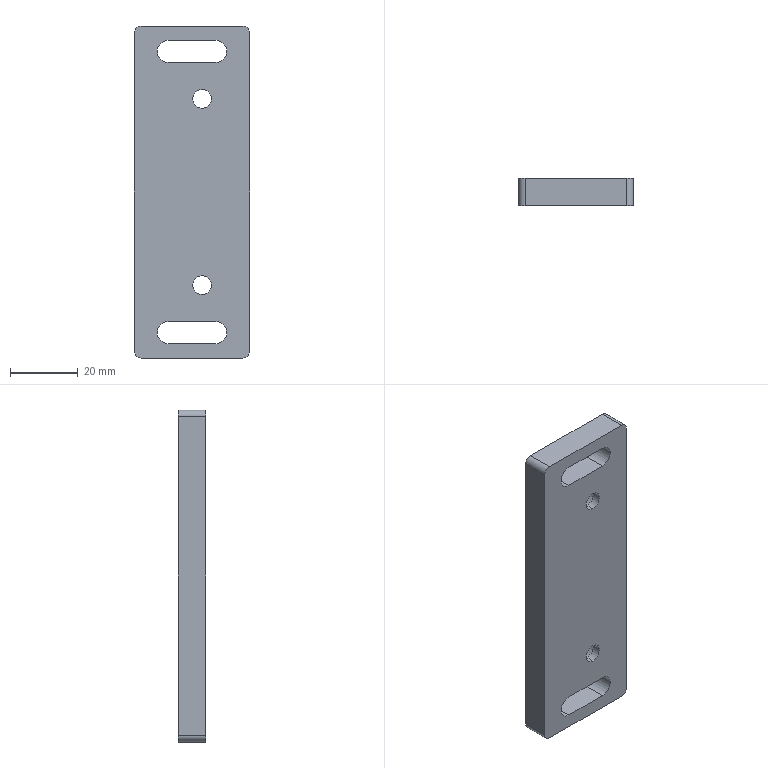Component | SolidWorks | PunchingKnifeBackingPlate.1-1 | 1 solid | 28 faces | box 34 x 8 x 98 mm | volume 23823 mm3 | cylinder 16 | plane 12 | commonest cylinder face diameters 9 x4 5.5 x4 4 x4 6.5 x4
build123d program:
from build123d import *

# Parameters (mm, degrees)
BOSS_EXTRUDE1_DEPTH                               = 8
HOLE_SIZE_ACCORDING_TO_TYPE_OF_HEX_SO_D           = 5.5
HOLE_SIZE_ACCORDING_TO_TYPE_OF_HEX_SO_CBORE_D     = 9
HOLE_SIZE_ACCORDING_TO_TYPE_OF_HEX_SO_CBORE_DEPTH = 5.5


with BuildPart() as part:
    # Sketch1 → Boss-Extrude1 (new body)
    with BuildSketch(Plane.XY):
        with BuildLine():
            Line((-47, 17), (47, 17))
            ThreePointArc((47, 17), (48.414, 16.414), (49, 15))
            Line((49, 15), (49, -15))
            ThreePointArc((49, -15), (48.414, -16.414), (47, -17))
            Line((47, -17), (-47, -17))
            ThreePointArc((-47, -17), (-48.414, -16.414), (-49, -15))
            Line((-49, -15), (-49, 15))
            ThreePointArc((-49, 15), (-48.414, 16.414), (-47, 17))
        make_face()
        with BuildLine():
            Line((-38.25, 7), (-38.25, -7))
            ThreePointArc((-38.25, -7), (-41.5, -10.25), (-44.75, -7))
            Line((-44.75, -7), (-44.75, 7))
            ThreePointArc((-44.75, 7), (-41.5, 10.25), (-38.25, 7))
        make_face(mode=Mode.SUBTRACT)
        with BuildLine():
            Line((44.75, 7), (44.75, -7))
            ThreePointArc((44.75, -7), (41.5, -10.25), (38.25, -7))
            Line((38.25, -7), (38.25, 7))
            ThreePointArc((38.25, 7), (41.5, 10.25), (44.75, 7))
        make_face(mode=Mode.SUBTRACT)
    extrude(amount=BOSS_EXTRUDE1_DEPTH)

    # Hole Size _ according to_ type of hex so (through all)
    with Locations(Plane.XY.offset(8)):
        with Locations((-27.5, 3), (27.5, 3)):
            CounterBoreHole(HOLE_SIZE_ACCORDING_TO_TYPE_OF_HEX_SO_D / 2, HOLE_SIZE_ACCORDING_TO_TYPE_OF_HEX_SO_CBORE_D / 2, HOLE_SIZE_ACCORDING_TO_TYPE_OF_HEX_SO_CBORE_DEPTH)


solid = part.part

# Placed as in the assembly
solid = solid.moved(Location((-25.75, 206, 0), (-90, 0, -90)))
STEP:
#1=COLOUR_RGB('',0.7922,0.8196,0.9333);
#2=FILL_AREA_STYLE_COLOUR('',#1);
#3=FILL_AREA_STYLE('',(#2));
#4=SURFACE_STYLE_FILL_AREA(#3);
#5=SURFACE_SIDE_STYLE('',(#4));
#6=SURFACE_STYLE_USAGE(.BOTH.,#5);
#7=PRESENTATION_STYLE_ASSIGNMENT((#6));
#8=CARTESIAN_POINT('',(-0.8957,8.209,-1.26));
#9=VERTEX_POINT('',#8);
#10=CARTESIAN_POINT('',(-0.8957,8.209,-0.9055));
#11=VERTEX_POINT('',#10);
#12=CARTESIAN_POINT('',(-0.8957,8.209,-1.083));
#13=DIRECTION('',(-0.,1.,0.));
#14=DIRECTION('',(0.,0.,1.));
#15=AXIS2_PLACEMENT_3D('',#12,#13,#14);
#16=CIRCLE('',#15,0.1772);
#17=EDGE_CURVE('',#9,#11,#16,.T.);
#18=ORIENTED_EDGE('',*,*,#17,.F.);
#19=CARTESIAN_POINT('',(-0.8957,8.425,-1.26));
#20=VERTEX_POINT('',#19);
#21=CARTESIAN_POINT('',(-0.8957,8.425,-1.26));
#22=DIRECTION('',(-0.,1.,0.));
#23=VECTOR('',#22,39.37);
#24=LINE('',#21,#23);
#25=EDGE_CURVE('',#9,#20,#24,.T.);
#26=ORIENTED_EDGE('',*,*,#25,.T.);
#27=CARTESIAN_POINT('',(-0.8957,8.425,-0.9055));
#28=VERTEX_POINT('',#27);
#29=CARTESIAN_POINT('',(-0.8957,8.425,-1.083));
#30=DIRECTION('',(-0.,1.,0.));
#31=DIRECTION('',(0.,0.,1.));
#32=AXIS2_PLACEMENT_3D('',#29,#30,#31);
#33=CIRCLE('',#32,0.1772);
#34=EDGE_CURVE('',#20,#28,#33,.T.);
#35=ORIENTED_EDGE('',*,*,#34,.T.);
#36=CARTESIAN_POINT('',(-0.8957,8.425,-0.9055));
#37=DIRECTION('',(-0.,1.,0.));
#38=VECTOR('',#37,39.37);
#39=LINE('',#36,#38);
#40=EDGE_CURVE('',#11,#28,#39,.T.);
#41=ORIENTED_EDGE('',*,*,#40,.F.);
#42=EDGE_LOOP('',(#18,#26,#35,#41));
#43=FACE_OUTER_BOUND('',#42,.T.);
#44=CARTESIAN_POINT('',(-0.8957,8.425,-1.083));
#45=DIRECTION('',(-0.,1.,0.));
#46=DIRECTION('',(0.,0.,1.));
#47=AXIS2_PLACEMENT_3D('',#44,#45,#46);
#48=CYLINDRICAL_SURFACE('',#47,0.1772);
#49=ADVANCED_FACE('',(#43),#48,.F.);
#50=CARTESIAN_POINT('',(-0.8957,8.11,-1.191));
#51=VERTEX_POINT('',#50);
#52=CARTESIAN_POINT('',(-0.8957,8.11,-0.9744));
#53=VERTEX_POINT('',#52);
#54=CARTESIAN_POINT('',(-0.8957,8.11,-1.083));
#55=DIRECTION('',(-0.,1.,0.));
#56=DIRECTION('',(0.,0.,1.));
#57=AXIS2_PLACEMENT_3D('',#54,#55,#56);
#58=CIRCLE('',#57,0.1083);
#59=EDGE_CURVE('',#51,#53,#58,.T.);
#60=ORIENTED_EDGE('',*,*,#59,.F.);
#61=CARTESIAN_POINT('',(-0.8957,8.209,-1.191));
#62=VERTEX_POINT('',#61);
#63=CARTESIAN_POINT('',(-0.8957,8.425,-1.191));
#64=DIRECTION('',(-0.,1.,0.));
#65=VECTOR('',#64,39.37);
#66=LINE('',#63,#65);
#67=EDGE_CURVE('',#51,#62,#66,.T.);
#68=ORIENTED_EDGE('',*,*,#67,.T.);
#69=CARTESIAN_POINT('',(-0.8957,8.209,-0.9744));
#70=VERTEX_POINT('',#69);
#71=CARTESIAN_POINT('',(-0.8957,8.209,-1.083));
#72=DIRECTION('',(-0.,1.,0.));
#73=DIRECTION('',(0.,0.,1.));
#74=AXIS2_PLACEMENT_3D('',#71,#72,#73);
#75=CIRCLE('',#74,0.1083);
#76=EDGE_CURVE('',#62,#70,#75,.T.);
#77=ORIENTED_EDGE('',*,*,#76,.T.);
#78=CARTESIAN_POINT('',(-0.8957,8.425,-0.9744));
#79=DIRECTION('',(-0.,1.,0.));
#80=VECTOR('',#79,39.37);
#81=LINE('',#78,#80);
#82=EDGE_CURVE('',#53,#70,#81,.T.);
#83=ORIENTED_EDGE('',*,*,#82,.F.);
#84=EDGE_LOOP('',(#60,#68,#77,#83));
#85=FACE_OUTER_BOUND('',#84,.T.);
#86=CARTESIAN_POINT('',(-0.8957,8.425,-1.083));
#87=DIRECTION('',(-0.,1.,0.));
#88=DIRECTION('',(0.,0.,1.));
#89=AXIS2_PLACEMENT_3D('',#86,#87,#88);
#90=CYLINDRICAL_SURFACE('',#89,0.1083);
#91=ADVANCED_FACE('',(#85),#90,.F.);
#92=CARTESIAN_POINT('',(-0.8957,8.209,0.9055));
#93=VERTEX_POINT('',#92);
#94=CARTESIAN_POINT('',(-0.8957,8.209,1.26));
#95=VERTEX_POINT('',#94);
#96=CARTESIAN_POINT('',(-0.8957,8.209,1.083));
#97=DIRECTION('',(-0.,1.,0.));
#98=DIRECTION('',(0.,0.,1.));
#99=AXIS2_PLACEMENT_3D('',#96,#97,#98);
#100=CIRCLE('',#99,0.1772);
#101=EDGE_CURVE('',#93,#95,#100,.T.);
#102=ORIENTED_EDGE('',*,*,#101,.F.);
#103=CARTESIAN_POINT('',(-0.8957,8.425,0.9055));
#104=VERTEX_POINT('',#103);
#105=CARTESIAN_POINT('',(-0.8957,8.425,0.9055));
#106=DIRECTION('',(-0.,1.,0.));
#107=VECTOR('',#106,39.37);
#108=LINE('',#105,#107);
#109=EDGE_CURVE('',#93,#104,#108,.T.);
#110=ORIENTED_EDGE('',*,*,#109,.T.);
#111=CARTESIAN_POINT('',(-0.8957,8.425,1.26));
#112=VERTEX_POINT('',#111);
#113=CARTESIAN_POINT('',(-0.8957,8.425,1.083));
#114=DIRECTION('',(-0.,1.,0.));
#115=DIRECTION('',(0.,0.,1.));
#116=AXIS2_PLACEMENT_3D('',#113,#114,#115);
#117=CIRCLE('',#116,0.1772);
#118=EDGE_CURVE('',#104,#112,#117,.T.);
#119=ORIENTED_EDGE('',*,*,#118,.T.);
#120=CARTESIAN_POINT('',(-0.8957,8.425,1.26));
#121=DIRECTION('',(-0.,1.,0.));
#122=VECTOR('',#121,39.37);
#123=LINE('',#120,#122);
#124=EDGE_CURVE('',#95,#112,#123,.T.);
#125=ORIENTED_EDGE('',*,*,#124,.F.);
#126=EDGE_LOOP('',(#102,#110,#119,#125));
#127=FACE_OUTER_BOUND('',#126,.T.);
#128=CARTESIAN_POINT('',(-0.8957,8.425,1.083));
#129=DIRECTION('',(-0.,1.,0.));
#130=DIRECTION('',(0.,0.,1.));
#131=AXIS2_PLACEMENT_3D('',#128,#129,#130);
#132=CYLINDRICAL_SURFACE('',#131,0.1772);
#133=ADVANCED_FACE('',(#127),#132,.F.);
#134=CARTESIAN_POINT('',(-0.8957,8.11,0.9744));
#135=VERTEX_POINT('',#134);
#136=CARTESIAN_POINT('',(-0.8957,8.11,1.191));
#137=VERTEX_POINT('',#136);
#138=CARTESIAN_POINT('',(-0.8957,8.11,1.083));
#139=DIRECTION('',(-0.,1.,0.));
#140=DIRECTION('',(0.,0.,1.));
#141=AXIS2_PLACEMENT_3D('',#138,#139,#140);
#142=CIRCLE('',#141,0.1083);
#143=EDGE_CURVE('',#135,#137,#142,.T.);
#144=ORIENTED_EDGE('',*,*,#143,.F.);
#145=CARTESIAN_POINT('',(-0.8957,8.209,0.9744));
#146=VERTEX_POINT('',#145);
#147=CARTESIAN_POINT('',(-0.8957,8.425,0.9744));
#148=DIRECTION('',(-0.,1.,0.));
#149=VECTOR('',#148,39.37);
#150=LINE('',#147,#149);
#151=EDGE_CURVE('',#135,#146,#150,.T.);
#152=ORIENTED_EDGE('',*,*,#151,.T.);
#153=CARTESIAN_POINT('',(-0.8957,8.209,1.191));
#154=VERTEX_POINT('',#153);
#155=CARTESIAN_POINT('',(-0.8957,8.209,1.083));
#156=DIRECTION('',(-0.,1.,0.));
#157=DIRECTION('',(0.,0.,1.));
#158=AXIS2_PLACEMENT_3D('',#155,#156,#157);
#159=CIRCLE('',#158,0.1083);
#160=EDGE_CURVE('',#146,#154,#159,.T.);
#161=ORIENTED_EDGE('',*,*,#160,.T.);
#162=CARTESIAN_POINT('',(-0.8957,8.425,1.191));
#163=DIRECTION('',(-0.,1.,0.));
#164=VECTOR('',#163,39.37);
#165=LINE('',#162,#164);
#166=EDGE_CURVE('',#137,#154,#165,.T.);
#167=ORIENTED_EDGE('',*,*,#166,.F.);
#168=EDGE_LOOP('',(#144,#152,#161,#167));
#169=FACE_OUTER_BOUND('',#168,.T.);
#170=CARTESIAN_POINT('',(-0.8957,8.425,1.083));
#171=DIRECTION('',(-0.,1.,0.));
#172=DIRECTION('',(0.,0.,1.));
#173=AXIS2_PLACEMENT_3D('',#170,#171,#172);
#174=CYLINDRICAL_SURFACE('',#173,0.1083);
#175=ADVANCED_FACE('',(#169),#174,.F.);
#176=CARTESIAN_POINT('',(-0.8957,8.425,-1.083));
#177=DIRECTION('',(-0.,1.,0.));
#178=DIRECTION('',(0.,0.,1.));
#179=AXIS2_PLACEMENT_3D('',#176,#177,#178);
#180=CIRCLE('',#179,0.1772);
#181=EDGE_CURVE('',#28,#20,#180,.T.);
#182=ORIENTED_EDGE('',*,*,#181,.F.);
#183=ORIENTED_EDGE('',*,*,#34,.F.);
#184=EDGE_LOOP('',(#182,#183));
#185=FACE_BOUND('',#184,.T.);
#186=CARTESIAN_POINT('',(-0.8957,8.425,1.083));
#187=DIRECTION('',(-0.,1.,0.));
#188=DIRECTION('',(0.,0.,1.));
#189=AXIS2_PLACEMENT_3D('',#186,#187,#188);
#190=CIRCLE('',#189,0.1772);
#191=EDGE_CURVE('',#112,#104,#190,.T.);
#192=ORIENTED_EDGE('',*,*,#191,.F.);
#193=ORIENTED_EDGE('',*,*,#118,.F.);
#194=EDGE_LOOP('',(#192,#193));
#195=FACE_BOUND('',#194,.T.);
#196=CARTESIAN_POINT('',(-0.7382,8.425,-1.762));
#197=VERTEX_POINT('',#196);
#198=CARTESIAN_POINT('',(-1.289,8.425,-1.762));
#199=VERTEX_POINT('',#198);
#200=CARTESIAN_POINT('',(-0.7382,8.425,-1.762));
#201=DIRECTION('',(-1.,-0.,0.));
#202=VECTOR('',#201,39.37);
#203=LINE('',#200,#202);
#204=EDGE_CURVE('',#197,#199,#203,.T.);
#205=ORIENTED_EDGE('',*,*,#204,.F.);
#206=CARTESIAN_POINT('',(-0.7382,8.425,-1.506));
#207=VERTEX_POINT('',#206);
#208=CARTESIAN_POINT('',(-0.7382,8.425,-1.634));
#209=DIRECTION('',(-0.,1.,0.));
#210=DIRECTION('',(0.,0.,1.));
#211=AXIS2_PLACEMENT_3D('',#208,#209,#210);
#212=CIRCLE('',#211,0.128);
#213=EDGE_CURVE('',#207,#197,#212,.T.);
#214=ORIENTED_EDGE('',*,*,#213,.F.);
#215=CARTESIAN_POINT('',(-1.289,8.425,-1.506));
#216=VERTEX_POINT('',#215);
#217=CARTESIAN_POINT('',(-0.7382,8.425,-1.506));
#218=DIRECTION('',(1.,0.,-0.));
#219=VECTOR('',#218,39.37);
#220=LINE('',#217,#219);
#221=EDGE_CURVE('',#216,#207,#220,.T.);
#222=ORIENTED_EDGE('',*,*,#221,.F.);
#223=CARTESIAN_POINT('',(-1.289,8.425,-1.634));
#224=DIRECTION('',(-0.,1.,0.));
#225=DIRECTION('',(0.,0.,1.));
#226=AXIS2_PLACEMENT_3D('',#223,#224,#225);
#227=CIRCLE('',#226,0.128);
#228=EDGE_CURVE('',#199,#216,#227,.T.);
#229=ORIENTED_EDGE('',*,*,#228,.F.);
#230=EDGE_LOOP('',(#205,#214,#222,#229));
#231=FACE_BOUND('',#230,.T.);
#232=CARTESIAN_POINT('',(-0.4232,8.425,1.929));
#233=VERTEX_POINT('',#232);
#234=CARTESIAN_POINT('',(-0.3445,8.425,1.85));
#235=VERTEX_POINT('',#234);
#236=CARTESIAN_POINT('',(-0.4232,8.425,1.85));
#237=DIRECTION('',(-0.,1.,0.));
#238=DIRECTION('',(0.,0.,1.));
#239=AXIS2_PLACEMENT_3D('',#236,#237,#238);
#240=CIRCLE('',#239,0.07874);
#241=EDGE_CURVE('',#233,#235,#240,.T.);
#242=ORIENTED_EDGE('',*,*,#241,.T.);
#243=CARTESIAN_POINT('',(-0.3445,8.425,-1.85));
#244=VERTEX_POINT('',#243);
#245=CARTESIAN_POINT('',(-0.3445,8.425,-1.85));
#246=DIRECTION('',(0.,-0.,-1.));
#247=VECTOR('',#246,39.37);
#248=LINE('',#245,#247);
#249=EDGE_CURVE('',#235,#244,#248,.T.);
#250=ORIENTED_EDGE('',*,*,#249,.T.);
#251=CARTESIAN_POINT('',(-0.4232,8.425,-1.929));
#252=VERTEX_POINT('',#251);
#253=CARTESIAN_POINT('',(-0.4232,8.425,-1.85));
#254=DIRECTION('',(-0.,1.,0.));
#255=DIRECTION('',(0.,0.,1.));
#256=AXIS2_PLACEMENT_3D('',#253,#254,#255);
#257=CIRCLE('',#256,0.07874);
#258=EDGE_CURVE('',#244,#252,#257,.T.);
#259=ORIENTED_EDGE('',*,*,#258,.T.);
#260=CARTESIAN_POINT('',(-1.604,8.425,-1.929));
#261=VERTEX_POINT('',#260);
#262=CARTESIAN_POINT('',(-0.4232,8.425,-1.929));
#263=DIRECTION('',(-1.,-0.,-0.));
#264=VECTOR('',#263,39.37);
#265=LINE('',#262,#264);
#266=EDGE_CURVE('',#252,#261,#265,.T.);
#267=ORIENTED_EDGE('',*,*,#266,.T.);
#268=CARTESIAN_POINT('',(-1.683,8.425,-1.85));
#269=VERTEX_POINT('',#268);
#270=CARTESIAN_POINT('',(-1.604,8.425,-1.85));
#271=DIRECTION('',(-0.,1.,0.));
#272=DIRECTION('',(0.,0.,-1.));
#273=AXIS2_PLACEMENT_3D('',#270,#271,#272);
#274=CIRCLE('',#273,0.07874);
#275=EDGE_CURVE('',#261,#269,#274,.T.);
#276=ORIENTED_EDGE('',*,*,#275,.T.);
#277=CARTESIAN_POINT('',(-1.683,8.425,1.85));
#278=VERTEX_POINT('',#277);
#279=CARTESIAN_POINT('',(-1.683,8.425,-1.85));
#280=DIRECTION('',(-0.,0.,1.));
#281=VECTOR('',#280,39.37);
#282=LINE('',#279,#281);
#283=EDGE_CURVE('',#269,#278,#282,.T.);
#284=ORIENTED_EDGE('',*,*,#283,.T.);
#285=CARTESIAN_POINT('',(-1.604,8.425,1.929));
#286=VERTEX_POINT('',#285);
#287=CARTESIAN_POINT('',(-1.604,8.425,1.85));
#288=DIRECTION('',(-0.,1.,0.));
#289=DIRECTION('',(0.,0.,-1.));
#290=AXIS2_PLACEMENT_3D('',#287,#288,#289);
#291=CIRCLE('',#290,0.07874);
#292=EDGE_CURVE('',#278,#286,#291,.T.);
#293=ORIENTED_EDGE('',*,*,#292,.T.);
#294=CARTESIAN_POINT('',(-0.4232,8.425,1.929));
#295=DIRECTION('',(1.,0.,0.));
#296=VECTOR('',#295,39.37);
#297=LINE('',#294,#296);
#298=EDGE_CURVE('',#286,#233,#297,.T.);
#299=ORIENTED_EDGE('',*,*,#298,.T.);
#300=EDGE_LOOP('',(#242,#250,#259,#267,#276,#284,#293,#299));
#301=FACE_OUTER_BOUND('',#300,.T.);
#302=CARTESIAN_POINT('',(-0.7382,8.425,1.506));
#303=VERTEX_POINT('',#302);
#304=CARTESIAN_POINT('',(-1.289,8.425,1.506));
#305=VERTEX_POINT('',#304);
#306=CARTESIAN_POINT('',(-0.7382,8.425,1.506));
#307=DIRECTION('',(-1.,-0.,-0.));
#308=VECTOR('',#307,39.37);
#309=LINE('',#306,#308);
#310=EDGE_CURVE('',#303,#305,#309,.T.);
#311=ORIENTED_EDGE('',*,*,#310,.F.);
#312=CARTESIAN_POINT('',(-0.7382,8.425,1.762));
#313=VERTEX_POINT('',#312);
#314=CARTESIAN_POINT('',(-0.7382,8.425,1.634));
#315=DIRECTION('',(-0.,1.,0.));
#316=DIRECTION('',(0.,0.,1.));
#317=AXIS2_PLACEMENT_3D('',#314,#315,#316);
#318=CIRCLE('',#317,0.128);
#319=EDGE_CURVE('',#313,#303,#318,.T.);
#320=ORIENTED_EDGE('',*,*,#319,.F.);
#321=CARTESIAN_POINT('',(-1.289,8.425,1.762));
#322=VERTEX_POINT('',#321);
#323=CARTESIAN_POINT('',(-0.7382,8.425,1.762));
#324=DIRECTION('',(1.,0.,0.));
#325=VECTOR('',#324,39.37);
#326=LINE('',#323,#325);
#327=EDGE_CURVE('',#322,#313,#326,.T.);
#328=ORIENTED_EDGE('',*,*,#327,.F.);
#329=CARTESIAN_POINT('',(-1.289,8.425,1.634));
#330=DIRECTION('',(-0.,1.,0.));
#331=DIRECTION('',(0.,0.,1.));
#332=AXIS2_PLACEMENT_3D('',#329,#330,#331);
#333=CIRCLE('',#332,0.128);
#334=EDGE_CURVE('',#305,#322,#333,.T.);
#335=ORIENTED_EDGE('',*,*,#334,.F.);
#336=EDGE_LOOP('',(#311,#320,#328,#335));
#337=FACE_BOUND('',#336,.T.);
#338=CARTESIAN_POINT('',(-0.4232,8.425,1.85));
#339=DIRECTION('',(-0.,1.,-0.));
#340=DIRECTION('',(-0.,0.,1.));
#341=AXIS2_PLACEMENT_3D('',#338,#339,#340);
#342=PLANE('',#341);
#343=ADVANCED_FACE('',(#185,#195,#231,#301,#337),#342,.T.);
#344=CARTESIAN_POINT('',(-0.8957,8.11,-1.083));
#345=DIRECTION('',(-0.,1.,0.));
#346=DIRECTION('',(0.,0.,1.));
#347=AXIS2_PLACEMENT_3D('',#344,#345,#346);
#348=CIRCLE('',#347,0.1083);
#349=EDGE_CURVE('',#53,#51,#348,.T.);
#350=ORIENTED_EDGE('',*,*,#349,.T.);
#351=ORIENTED_EDGE('',*,*,#59,.T.);
#352=EDGE_LOOP('',(#350,#351));
#353=FACE_BOUND('',#352,.T.);
#354=CARTESIAN_POINT('',(-0.8957,8.11,1.083));
#355=DIRECTION('',(-0.,1.,0.));
#356=DIRECTION('',(0.,0.,1.));
#357=AXIS2_PLACEMENT_3D('',#354,#355,#356);
#358=CIRCLE('',#357,0.1083);
#359=EDGE_CURVE('',#137,#135,#358,.T.);
#360=ORIENTED_EDGE('',*,*,#359,.T.);
#361=ORIENTED_EDGE('',*,*,#143,.T.);
#362=EDGE_LOOP('',(#360,#361));
#363=FACE_BOUND('',#362,.T.);
#364=CARTESIAN_POINT('',(-0.7382,8.11,-1.506));
#365=VERTEX_POINT('',#364);
#366=CARTESIAN_POINT('',(-0.7382,8.11,-1.762));
#367=VERTEX_POINT('',#366);
#368=CARTESIAN_POINT('',(-0.7382,8.11,-1.634));
#369=DIRECTION('',(-0.,1.,0.));
#370=DIRECTION('',(0.,0.,1.));
#371=AXIS2_PLACEMENT_3D('',#368,#369,#370);
#372=CIRCLE('',#371,0.128);
#373=EDGE_CURVE('',#365,#367,#372,.T.);
#374=ORIENTED_EDGE('',*,*,#373,.T.);
#375=CARTESIAN_POINT('',(-1.289,8.11,-1.762));
#376=VERTEX_POINT('',#375);
#377=CARTESIAN_POINT('',(-0.7382,8.11,-1.762));
#378=DIRECTION('',(-1.,-0.,0.));
#379=VECTOR('',#378,39.37);
#380=LINE('',#377,#379);
#381=EDGE_CURVE('',#367,#376,#380,.T.);
#382=ORIENTED_EDGE('',*,*,#381,.T.);
#383=CARTESIAN_POINT('',(-1.289,8.11,-1.506));
#384=VERTEX_POINT('',#383);
#385=CARTESIAN_POINT('',(-1.289,8.11,-1.634));
#386=DIRECTION('',(-0.,1.,0.));
#387=DIRECTION('',(0.,0.,1.));
#388=AXIS2_PLACEMENT_3D('',#385,#386,#387);
#389=CIRCLE('',#388,0.128);
#390=EDGE_CURVE('',#376,#384,#389,.T.);
#391=ORIENTED_EDGE('',*,*,#390,.T.);
#392=CARTESIAN_POINT('',(-0.7382,8.11,-1.506));
#393=DIRECTION('',(1.,0.,-0.));
#394=VECTOR('',#393,39.37);
#395=LINE('',#392,#394);
#396=EDGE_CURVE('',#384,#365,#395,.T.);
#397=ORIENTED_EDGE('',*,*,#396,.T.);
#398=EDGE_LOOP('',(#374,#382,#391,#397));
#399=FACE_BOUND('',#398,.T.);
#400=CARTESIAN_POINT('',(-0.4232,8.11,1.929));
#401=VERTEX_POINT('',#400);
#402=CARTESIAN_POINT('',(-0.3445,8.11,1.85));
#403=VERTEX_POINT('',#402);
#404=CARTESIAN_POINT('',(-0.4232,8.11,1.85));
#405=DIRECTION('',(-0.,1.,0.));
#406=DIRECTION('',(0.,0.,1.));
#407=AXIS2_PLACEMENT_3D('',#404,#405,#406);
#408=CIRCLE('',#407,0.07874);
#409=EDGE_CURVE('',#401,#403,#408,.T.);
#410=ORIENTED_EDGE('',*,*,#409,.F.);
#411=CARTESIAN_POINT('',(-1.604,8.11,1.929));
#412=VERTEX_POINT('',#411);
#413=CARTESIAN_POINT('',(-0.4232,8.11,1.929));
#414=DIRECTION('',(1.,0.,0.));
#415=VECTOR('',#414,39.37);
#416=LINE('',#413,#415);
#417=EDGE_CURVE('',#412,#401,#416,.T.);
#418=ORIENTED_EDGE('',*,*,#417,.F.);
#419=CARTESIAN_POINT('',(-1.683,8.11,1.85));
#420=VERTEX_POINT('',#419);
#421=CARTESIAN_POINT('',(-1.604,8.11,1.85));
#422=DIRECTION('',(-0.,1.,0.));
#423=DIRECTION('',(0.,0.,-1.));
#424=AXIS2_PLACEMENT_3D('',#421,#422,#423);
#425=CIRCLE('',#424,0.07874);
#426=EDGE_CURVE('',#420,#412,#425,.T.);
#427=ORIENTED_EDGE('',*,*,#426,.F.);
#428=CARTESIAN_POINT('',(-1.683,8.11,-1.85));
#429=VERTEX_POINT('',#428);
#430=CARTESIAN_POINT('',(-1.683,8.11,-1.85));
#431=DIRECTION('',(-0.,0.,1.));
#432=VECTOR('',#431,39.37);
#433=LINE('',#430,#432);
#434=EDGE_CURVE('',#429,#420,#433,.T.);
#435=ORIENTED_EDGE('',*,*,#434,.F.);
#436=CARTESIAN_POINT('',(-1.604,8.11,-1.929));
#437=VERTEX_POINT('',#436);
#438=CARTESIAN_POINT('',(-1.604,8.11,-1.85));
#439=DIRECTION('',(-0.,1.,0.));
#440=DIRECTION('',(0.,0.,-1.));
#441=AXIS2_PLACEMENT_3D('',#438,#439,#440);
#442=CIRCLE('',#441,0.07874);
#443=EDGE_CURVE('',#437,#429,#442,.T.);
#444=ORIENTED_EDGE('',*,*,#443,.F.);
#445=CARTESIAN_POINT('',(-0.4232,8.11,-1.929));
#446=VERTEX_POINT('',#445);
#447=CARTESIAN_POINT('',(-0.4232,8.11,-1.929));
#448=DIRECTION('',(-1.,-0.,-0.));
#449=VECTOR('',#448,39.37);
#450=LINE('',#447,#449);
#451=EDGE_CURVE('',#446,#437,#450,.T.);
#452=ORIENTED_EDGE('',*,*,#451,.F.);
#453=CARTESIAN_POINT('',(-0.3445,8.11,-1.85));
#454=VERTEX_POINT('',#453);
#455=CARTESIAN_POINT('',(-0.4232,8.11,-1.85));
#456=DIRECTION('',(-0.,1.,0.));
#457=DIRECTION('',(0.,0.,1.));
#458=AXIS2_PLACEMENT_3D('',#455,#456,#457);
#459=CIRCLE('',#458,0.07874);
#460=EDGE_CURVE('',#454,#446,#459,.T.);
#461=ORIENTED_EDGE('',*,*,#460,.F.);
#462=CARTESIAN_POINT('',(-0.3445,8.11,-1.85));
#463=DIRECTION('',(0.,-0.,-1.));
#464=VECTOR('',#463,39.37);
#465=LINE('',#462,#464);
#466=EDGE_CURVE('',#403,#454,#465,.T.);
#467=ORIENTED_EDGE('',*,*,#466,.F.);
#468=EDGE_LOOP('',(#410,#418,#427,#435,#444,#452,#461,#467));
#469=FACE_OUTER_BOUND('',#468,.T.);
#470=CARTESIAN_POINT('',(-0.7382,8.11,1.762));
#471=VERTEX_POINT('',#470);
#472=CARTESIAN_POINT('',(-0.7382,8.11,1.506));
#473=VERTEX_POINT('',#472);
#474=CARTESIAN_POINT('',(-0.7382,8.11,1.634));
#475=DIRECTION('',(-0.,1.,0.));
#476=DIRECTION('',(0.,0.,1.));
#477=AXIS2_PLACEMENT_3D('',#474,#475,#476);
#478=CIRCLE('',#477,0.128);
#479=EDGE_CURVE('',#471,#473,#478,.T.);
#480=ORIENTED_EDGE('',*,*,#479,.T.);
#481=CARTESIAN_POINT('',(-1.289,8.11,1.506));
#482=VERTEX_POINT('',#481);
#483=CARTESIAN_POINT('',(-0.7382,8.11,1.506));
#484=DIRECTION('',(-1.,-0.,-0.));
#485=VECTOR('',#484,39.37);
#486=LINE('',#483,#485);
#487=EDGE_CURVE('',#473,#482,#486,.T.);
#488=ORIENTED_EDGE('',*,*,#487,.T.);
#489=CARTESIAN_POINT('',(-1.289,8.11,1.762));
#490=VERTEX_POINT('',#489);
#491=CARTESIAN_POINT('',(-1.289,8.11,1.634));
#492=DIRECTION('',(-0.,1.,0.));
#493=DIRECTION('',(0.,0.,1.));
#494=AXIS2_PLACEMENT_3D('',#491,#492,#493);
#495=CIRCLE('',#494,0.128);
#496=EDGE_CURVE('',#482,#490,#495,.T.);
#497=ORIENTED_EDGE('',*,*,#496,.T.);
#498=CARTESIAN_POINT('',(-0.7382,8.11,1.762));
#499=DIRECTION('',(1.,0.,0.));
#500=VECTOR('',#499,39.37);
#501=LINE('',#498,#500);
#502=EDGE_CURVE('',#490,#471,#501,.T.);
#503=ORIENTED_EDGE('',*,*,#502,.T.);
#504=EDGE_LOOP('',(#480,#488,#497,#503));
#505=FACE_BOUND('',#504,.T.);
#506=CARTESIAN_POINT('',(-0.4232,8.11,1.85));
#507=DIRECTION('',(-0.,1.,-0.));
#508=DIRECTION('',(-0.,0.,1.));
#509=AXIS2_PLACEMENT_3D('',#506,#507,#508);
#510=PLANE('',#509);
#511=ADVANCED_FACE('',(#353,#363,#399,#469,#505),#510,.F.);
#512=ORIENTED_EDGE('',*,*,#409,.T.);
#513=CARTESIAN_POINT('',(-0.3445,8.425,1.85));
#514=DIRECTION('',(0.,-1.,-0.));
#515=VECTOR('',#514,39.37);
#516=LINE('',#513,#515);
#517=EDGE_CURVE('',#235,#403,#516,.T.);
#518=ORIENTED_EDGE('',*,*,#517,.F.);
#519=ORIENTED_EDGE('',*,*,#241,.F.);
#520=CARTESIAN_POINT('',(-0.4232,8.425,1.929));
#521=DIRECTION('',(0.,-1.,-0.));
#522=VECTOR('',#521,39.37);
#523=LINE('',#520,#522);
#524=EDGE_CURVE('',#233,#401,#523,.T.);
#525=ORIENTED_EDGE('',*,*,#524,.T.);
#526=EDGE_LOOP('',(#512,#518,#519,#525));
#527=FACE_OUTER_BOUND('',#526,.T.);
#528=CARTESIAN_POINT('',(-0.4232,8.425,1.85));
#529=DIRECTION('',(0.,-1.,-0.));
#530=DIRECTION('',(0.,0.,-1.));
#531=AXIS2_PLACEMENT_3D('',#528,#529,#530);
#532=CYLINDRICAL_SURFACE('',#531,0.07874);
#533=ADVANCED_FACE('',(#527),#532,.T.);
#534=ORIENTED_EDGE('',*,*,#466,.T.);
#535=CARTESIAN_POINT('',(-0.3445,8.425,-1.85));
#536=DIRECTION('',(0.,-1.,-0.));
#537=VECTOR('',#536,39.37);
#538=LINE('',#535,#537);
#539=EDGE_CURVE('',#244,#454,#538,.T.);
#540=ORIENTED_EDGE('',*,*,#539,.F.);
#541=ORIENTED_EDGE('',*,*,#249,.F.);
#542=ORIENTED_EDGE('',*,*,#517,.T.);
#543=EDGE_LOOP('',(#534,#540,#541,#542));
#544=FACE_OUTER_BOUND('',#543,.T.);
#545=CARTESIAN_POINT('',(-0.3445,8.425,-1.85));
#546=DIRECTION('',(-1.,-0.,-0.));
#547=DIRECTION('',(0.,-1.,-0.));
#548=AXIS2_PLACEMENT_3D('',#545,#546,#547);
#549=PLANE('',#548);
#550=ADVANCED_FACE('',(#544),#549,.F.);
#551=ORIENTED_EDGE('',*,*,#460,.T.);
#552=CARTESIAN_POINT('',(-0.4232,8.425,-1.929));
#553=DIRECTION('',(0.,-1.,-0.));
#554=VECTOR('',#553,39.37);
#555=LINE('',#552,#554);
#556=EDGE_CURVE('',#252,#446,#555,.T.);
#557=ORIENTED_EDGE('',*,*,#556,.F.);
#558=ORIENTED_EDGE('',*,*,#258,.F.);
#559=ORIENTED_EDGE('',*,*,#539,.T.);
#560=EDGE_LOOP('',(#551,#557,#558,#559));
#561=FACE_OUTER_BOUND('',#560,.T.);
#562=CARTESIAN_POINT('',(-0.4232,8.425,-1.85));
#563=DIRECTION('',(0.,-1.,-0.));
#564=DIRECTION('',(0.,0.,-1.));
#565=AXIS2_PLACEMENT_3D('',#562,#563,#564);
#566=CYLINDRICAL_SURFACE('',#565,0.07874);
#567=ADVANCED_FACE('',(#561),#566,.T.);
#568=ORIENTED_EDGE('',*,*,#451,.T.);
#569=CARTESIAN_POINT('',(-1.604,8.425,-1.929));
#570=DIRECTION('',(0.,-1.,-0.));
#571=VECTOR('',#570,39.37);
#572=LINE('',#569,#571);
#573=EDGE_CURVE('',#261,#437,#572,.T.);
#574=ORIENTED_EDGE('',*,*,#573,.F.);
#575=ORIENTED_EDGE('',*,*,#266,.F.);
#576=ORIENTED_EDGE('',*,*,#556,.T.);
#577=EDGE_LOOP('',(#568,#574,#575,#576));
#578=FACE_OUTER_BOUND('',#577,.T.);
#579=CARTESIAN_POINT('',(-0.4232,8.425,-1.929));
#580=DIRECTION('',(-0.,-0.,1.));
#581=DIRECTION('',(0.,-1.,-0.));
#582=AXIS2_PLACEMENT_3D('',#579,#580,#581);
#583=PLANE('',#582);
#584=ADVANCED_FACE('',(#578),#583,.F.);
#585=ORIENTED_EDGE('',*,*,#443,.T.);
#586=CARTESIAN_POINT('',(-1.683,8.425,-1.85));
#587=DIRECTION('',(0.,-1.,-0.));
#588=VECTOR('',#587,39.37);
#589=LINE('',#586,#588);
#590=EDGE_CURVE('',#269,#429,#589,.T.);
#591=ORIENTED_EDGE('',*,*,#590,.F.);
#592=ORIENTED_EDGE('',*,*,#275,.F.);
#593=ORIENTED_EDGE('',*,*,#573,.T.);
#594=EDGE_LOOP('',(#585,#591,#592,#593));
#595=FACE_OUTER_BOUND('',#594,.T.);
#596=CARTESIAN_POINT('',(-1.604,8.425,-1.85));
#597=DIRECTION('',(0.,-1.,-0.));
#598=DIRECTION('',(0.,0.,-1.));
#599=AXIS2_PLACEMENT_3D('',#596,#597,#598);
#600=CYLINDRICAL_SURFACE('',#599,0.07874);
#601=ADVANCED_FACE('',(#595),#600,.T.);
#602=ORIENTED_EDGE('',*,*,#434,.T.);
#603=CARTESIAN_POINT('',(-1.683,8.425,1.85));
#604=DIRECTION('',(0.,-1.,-0.));
#605=VECTOR('',#604,39.37);
#606=LINE('',#603,#605);
#607=EDGE_CURVE('',#278,#420,#606,.T.);
#608=ORIENTED_EDGE('',*,*,#607,.F.);
#609=ORIENTED_EDGE('',*,*,#283,.F.);
#610=ORIENTED_EDGE('',*,*,#590,.T.);
#611=EDGE_LOOP('',(#602,#608,#609,#610));
#612=FACE_OUTER_BOUND('',#611,.T.);
#613=CARTESIAN_POINT('',(-1.683,8.425,-1.85));
#614=DIRECTION('',(1.,0.,0.));
#615=DIRECTION('',(0.,-0.,-1.));
#616=AXIS2_PLACEMENT_3D('',#613,#614,#615);
#617=PLANE('',#616);
#618=ADVANCED_FACE('',(#612),#617,.F.);
#619=ORIENTED_EDGE('',*,*,#426,.T.);
#620=CARTESIAN_POINT('',(-1.604,8.425,1.929));
#621=DIRECTION('',(0.,-1.,-0.));
#622=VECTOR('',#621,39.37);
#623=LINE('',#620,#622);
#624=EDGE_CURVE('',#286,#412,#623,.T.);
#625=ORIENTED_EDGE('',*,*,#624,.F.);
#626=ORIENTED_EDGE('',*,*,#292,.F.);
#627=ORIENTED_EDGE('',*,*,#607,.T.);
#628=EDGE_LOOP('',(#619,#625,#626,#627));
#629=FACE_OUTER_BOUND('',#628,.T.);
#630=CARTESIAN_POINT('',(-1.604,8.425,1.85));
#631=DIRECTION('',(0.,-1.,-0.));
#632=DIRECTION('',(0.,0.,-1.));
#633=AXIS2_PLACEMENT_3D('',#630,#631,#632);
#634=CYLINDRICAL_SURFACE('',#633,0.07874);
#635=ADVANCED_FACE('',(#629),#634,.T.);
#636=ORIENTED_EDGE('',*,*,#417,.T.);
#637=ORIENTED_EDGE('',*,*,#524,.F.);
#638=ORIENTED_EDGE('',*,*,#298,.F.);
#639=ORIENTED_EDGE('',*,*,#624,.T.);
#640=EDGE_LOOP('',(#636,#637,#638,#639));
#641=FACE_OUTER_BOUND('',#640,.T.);
#642=CARTESIAN_POINT('',(-0.4232,8.425,1.929));
#643=DIRECTION('',(0.,0.,-1.));
#644=DIRECTION('',(-0.,1.,0.));
#645=AXIS2_PLACEMENT_3D('',#642,#643,#644);
#646=PLANE('',#645);
#647=ADVANCED_FACE('',(#641),#646,.F.);
#648=ORIENTED_EDGE('',*,*,#373,.F.);
#649=CARTESIAN_POINT('',(-0.7382,8.425,-1.506));
#650=DIRECTION('',(0.,-1.,-0.));
#651=VECTOR('',#650,39.37);
#652=LINE('',#649,#651);
#653=EDGE_CURVE('',#207,#365,#652,.T.);
#654=ORIENTED_EDGE('',*,*,#653,.F.);
#655=ORIENTED_EDGE('',*,*,#213,.T.);
#656=CARTESIAN_POINT('',(-0.7382,8.425,-1.762));
#657=DIRECTION('',(0.,-1.,-0.));
#658=VECTOR('',#657,39.37);
#659=LINE('',#656,#658);
#660=EDGE_CURVE('',#197,#367,#659,.T.);
#661=ORIENTED_EDGE('',*,*,#660,.T.);
#662=EDGE_LOOP('',(#648,#654,#655,#661));
#663=FACE_OUTER_BOUND('',#662,.T.);
#664=CARTESIAN_POINT('',(-0.7382,8.425,-1.634));
#665=DIRECTION('',(0.,-1.,-0.));
#666=DIRECTION('',(0.,0.,-1.));
#667=AXIS2_PLACEMENT_3D('',#664,#665,#666);
#668=CYLINDRICAL_SURFACE('',#667,0.128);
#669=ADVANCED_FACE('',(#663),#668,.F.);
#670=ORIENTED_EDGE('',*,*,#381,.F.);
#671=ORIENTED_EDGE('',*,*,#660,.F.);
#672=ORIENTED_EDGE('',*,*,#204,.T.);
#673=CARTESIAN_POINT('',(-1.289,8.425,-1.762));
#674=DIRECTION('',(0.,-1.,-0.));
#675=VECTOR('',#674,39.37);
#676=LINE('',#673,#675);
#677=EDGE_CURVE('',#199,#376,#676,.T.);
#678=ORIENTED_EDGE('',*,*,#677,.T.);
#679=EDGE_LOOP('',(#670,#671,#672,#678));
#680=FACE_OUTER_BOUND('',#679,.T.);
#681=CARTESIAN_POINT('',(-0.7382,8.425,-1.762));
#682=DIRECTION('',(0.,0.,1.));
#683=DIRECTION('',(1.,0.,-0.));
#684=AXIS2_PLACEMENT_3D('',#681,#682,#683);
#685=PLANE('',#684);
#686=ADVANCED_FACE('',(#680),#685,.T.);
#687=ORIENTED_EDGE('',*,*,#390,.F.);
#688=ORIENTED_EDGE('',*,*,#677,.F.);
#689=ORIENTED_EDGE('',*,*,#228,.T.);
#690=CARTESIAN_POINT('',(-1.289,8.425,-1.506));
#691=DIRECTION('',(0.,-1.,-0.));
#692=VECTOR('',#691,39.37);
#693=LINE('',#690,#692);
#694=EDGE_CURVE('',#216,#384,#693,.T.);
#695=ORIENTED_EDGE('',*,*,#694,.T.);
#696=EDGE_LOOP('',(#687,#688,#689,#695));
#697=FACE_OUTER_BOUND('',#696,.T.);
#698=CARTESIAN_POINT('',(-1.289,8.425,-1.634));
#699=DIRECTION('',(0.,-1.,-0.));
#700=DIRECTION('',(0.,0.,-1.));
#701=AXIS2_PLACEMENT_3D('',#698,#699,#700);
#702=CYLINDRICAL_SURFACE('',#701,0.128);
#703=ADVANCED_FACE('',(#697),#702,.F.);
#704=ORIENTED_EDGE('',*,*,#396,.F.);
#705=ORIENTED_EDGE('',*,*,#694,.F.);
#706=ORIENTED_EDGE('',*,*,#221,.T.);
#707=ORIENTED_EDGE('',*,*,#653,.T.);
#708=EDGE_LOOP('',(#704,#705,#706,#707));
#709=FACE_OUTER_BOUND('',#708,.T.);
#710=CARTESIAN_POINT('',(-0.7382,8.425,-1.506));
#711=DIRECTION('',(-0.,-0.,-1.));
#712=DIRECTION('',(-1.,-0.,0.));
#713=AXIS2_PLACEMENT_3D('',#710,#711,#712);
#714=PLANE('',#713);
#715=ADVANCED_FACE('',(#709),#714,.T.);
#716=ORIENTED_EDGE('',*,*,#479,.F.);
#717=CARTESIAN_POINT('',(-0.7382,8.425,1.762));
#718=DIRECTION('',(0.,-1.,-0.));
#719=VECTOR('',#718,39.37);
#720=LINE('',#717,#719);
#721=EDGE_CURVE('',#313,#471,#720,.T.);
#722=ORIENTED_EDGE('',*,*,#721,.F.);
#723=ORIENTED_EDGE('',*,*,#319,.T.);
#724=CARTESIAN_POINT('',(-0.7382,8.425,1.506));
#725=DIRECTION('',(0.,-1.,-0.));
#726=VECTOR('',#725,39.37);
#727=LINE('',#724,#726);
#728=EDGE_CURVE('',#303,#473,#727,.T.);
#729=ORIENTED_EDGE('',*,*,#728,.T.);
#730=EDGE_LOOP('',(#716,#722,#723,#729));
#731=FACE_OUTER_BOUND('',#730,.T.);
#732=CARTESIAN_POINT('',(-0.7382,8.425,1.634));
#733=DIRECTION('',(0.,-1.,-0.));
#734=DIRECTION('',(0.,0.,-1.));
#735=AXIS2_PLACEMENT_3D('',#732,#733,#734);
#736=CYLINDRICAL_SURFACE('',#735,0.128);
#737=ADVANCED_FACE('',(#731),#736,.F.);
#738=ORIENTED_EDGE('',*,*,#487,.F.);
#739=ORIENTED_EDGE('',*,*,#728,.F.);
#740=ORIENTED_EDGE('',*,*,#310,.T.);
#741=CARTESIAN_POINT('',(-1.289,8.425,1.506));
#742=DIRECTION('',(0.,-1.,-0.));
#743=VECTOR('',#742,39.37);
#744=LINE('',#741,#743);
#745=EDGE_CURVE('',#305,#482,#744,.T.);
#746=ORIENTED_EDGE('',*,*,#745,.T.);
#747=EDGE_LOOP('',(#738,#739,#740,#746));
#748=FACE_OUTER_BOUND('',#747,.T.);
#749=CARTESIAN_POINT('',(-0.7382,8.425,1.506));
#750=DIRECTION('',(-0.,-0.,1.));
#751=DIRECTION('',(0.,-1.,-0.));
#752=AXIS2_PLACEMENT_3D('',#749,#750,#751);
#753=PLANE('',#752);
#754=ADVANCED_FACE('',(#748),#753,.T.);
#755=ORIENTED_EDGE('',*,*,#496,.F.);
#756=ORIENTED_EDGE('',*,*,#745,.F.);
#757=ORIENTED_EDGE('',*,*,#334,.T.);
#758=CARTESIAN_POINT('',(-1.289,8.425,1.762));
#759=DIRECTION('',(0.,-1.,-0.));
#760=VECTOR('',#759,39.37);
#761=LINE('',#758,#760);
#762=EDGE_CURVE('',#322,#490,#761,.T.);
#763=ORIENTED_EDGE('',*,*,#762,.T.);
#764=EDGE_LOOP('',(#755,#756,#757,#763));
#765=FACE_OUTER_BOUND('',#764,.T.);
#766=CARTESIAN_POINT('',(-1.289,8.425,1.634));
#767=DIRECTION('',(0.,-1.,-0.));
#768=DIRECTION('',(0.,0.,-1.));
#769=AXIS2_PLACEMENT_3D('',#766,#767,#768);
#770=CYLINDRICAL_SURFACE('',#769,0.128);
#771=ADVANCED_FACE('',(#765),#770,.F.);
#772=ORIENTED_EDGE('',*,*,#502,.F.);
#773=ORIENTED_EDGE('',*,*,#762,.F.);
#774=ORIENTED_EDGE('',*,*,#327,.T.);
#775=ORIENTED_EDGE('',*,*,#721,.T.);
#776=EDGE_LOOP('',(#772,#773,#774,#775));
#777=FACE_OUTER_BOUND('',#776,.T.);
#778=CARTESIAN_POINT('',(-0.7382,8.425,1.762));
#779=DIRECTION('',(0.,0.,-1.));
#780=DIRECTION('',(-0.,1.,0.));
#781=AXIS2_PLACEMENT_3D('',#778,#779,#780);
#782=PLANE('',#781);
#783=ADVANCED_FACE('',(#777),#782,.T.);
#784=ORIENTED_EDGE('',*,*,#151,.F.);
#785=ORIENTED_EDGE('',*,*,#359,.F.);
#786=ORIENTED_EDGE('',*,*,#166,.T.);
#787=CARTESIAN_POINT('',(-0.8957,8.209,1.083));
#788=DIRECTION('',(-0.,1.,0.));
#789=DIRECTION('',(0.,0.,1.));
#790=AXIS2_PLACEMENT_3D('',#787,#788,#789);
#791=CIRCLE('',#790,0.1083);
#792=EDGE_CURVE('',#154,#146,#791,.T.);
#793=ORIENTED_EDGE('',*,*,#792,.T.);
#794=EDGE_LOOP('',(#784,#785,#786,#793));
#795=FACE_OUTER_BOUND('',#794,.T.);
#796=CARTESIAN_POINT('',(-0.8957,8.425,1.083));
#797=DIRECTION('',(-0.,1.,0.));
#798=DIRECTION('',(0.,0.,1.));
#799=AXIS2_PLACEMENT_3D('',#796,#797,#798);
#800=CYLINDRICAL_SURFACE('',#799,0.1083);
#801=ADVANCED_FACE('',(#795),#800,.F.);
#802=ORIENTED_EDGE('',*,*,#792,.F.);
#803=ORIENTED_EDGE('',*,*,#160,.F.);
#804=EDGE_LOOP('',(#802,#803));
#805=FACE_BOUND('',#804,.T.);
#806=CARTESIAN_POINT('',(-0.8957,8.209,1.083));
#807=DIRECTION('',(-0.,1.,0.));
#808=DIRECTION('',(0.,0.,1.));
#809=AXIS2_PLACEMENT_3D('',#806,#807,#808);
#810=CIRCLE('',#809,0.1772);
#811=EDGE_CURVE('',#95,#93,#810,.T.);
#812=ORIENTED_EDGE('',*,*,#811,.T.);
#813=ORIENTED_EDGE('',*,*,#101,.T.);
#814=EDGE_LOOP('',(#812,#813));
#815=FACE_OUTER_BOUND('',#814,.T.);
#816=CARTESIAN_POINT('',(-0.8957,8.209,1.191));
#817=DIRECTION('',(0.,-1.,0.));
#818=DIRECTION('',(0.,-0.,-1.));
#819=AXIS2_PLACEMENT_3D('',#816,#817,#818);
#820=PLANE('',#819);
#821=ADVANCED_FACE('',(#805,#815),#820,.F.);
#822=ORIENTED_EDGE('',*,*,#109,.F.);
#823=ORIENTED_EDGE('',*,*,#811,.F.);
#824=ORIENTED_EDGE('',*,*,#124,.T.);
#825=ORIENTED_EDGE('',*,*,#191,.T.);
#826=EDGE_LOOP('',(#822,#823,#824,#825));
#827=FACE_OUTER_BOUND('',#826,.T.);
#828=CARTESIAN_POINT('',(-0.8957,8.425,1.083));
#829=DIRECTION('',(-0.,1.,0.));
#830=DIRECTION('',(0.,0.,1.));
#831=AXIS2_PLACEMENT_3D('',#828,#829,#830);
#832=CYLINDRICAL_SURFACE('',#831,0.1772);
#833=ADVANCED_FACE('',(#827),#832,.F.);
#834=ORIENTED_EDGE('',*,*,#67,.F.);
#835=ORIENTED_EDGE('',*,*,#349,.F.);
#836=ORIENTED_EDGE('',*,*,#82,.T.);
#837=CARTESIAN_POINT('',(-0.8957,8.209,-1.083));
#838=DIRECTION('',(-0.,1.,0.));
#839=DIRECTION('',(0.,0.,1.));
#840=AXIS2_PLACEMENT_3D('',#837,#838,#839);
#841=CIRCLE('',#840,0.1083);
#842=EDGE_CURVE('',#70,#62,#841,.T.);
#843=ORIENTED_EDGE('',*,*,#842,.T.);
#844=EDGE_LOOP('',(#834,#835,#836,#843));
#845=FACE_OUTER_BOUND('',#844,.T.);
#846=CARTESIAN_POINT('',(-0.8957,8.425,-1.083));
#847=DIRECTION('',(-0.,1.,0.));
#848=DIRECTION('',(0.,0.,1.));
#849=AXIS2_PLACEMENT_3D('',#846,#847,#848);
#850=CYLINDRICAL_SURFACE('',#849,0.1083);
#851=ADVANCED_FACE('',(#845),#850,.F.);
#852=ORIENTED_EDGE('',*,*,#842,.F.);
#853=ORIENTED_EDGE('',*,*,#76,.F.);
#854=EDGE_LOOP('',(#852,#853));
#855=FACE_BOUND('',#854,.T.);
#856=CARTESIAN_POINT('',(-0.8957,8.209,-1.083));
#857=DIRECTION('',(-0.,1.,0.));
#858=DIRECTION('',(0.,0.,1.));
#859=AXIS2_PLACEMENT_3D('',#856,#857,#858);
#860=CIRCLE('',#859,0.1772);
#861=EDGE_CURVE('',#11,#9,#860,.T.);
#862=ORIENTED_EDGE('',*,*,#861,.T.);
#863=ORIENTED_EDGE('',*,*,#17,.T.);
#864=EDGE_LOOP('',(#862,#863));
#865=FACE_OUTER_BOUND('',#864,.T.);
#866=CARTESIAN_POINT('',(-0.8957,8.209,-0.9744));
#867=DIRECTION('',(0.,-1.,0.));
#868=DIRECTION('',(0.,-0.,-1.));
#869=AXIS2_PLACEMENT_3D('',#866,#867,#868);
#870=PLANE('',#869);
#871=ADVANCED_FACE('',(#855,#865),#870,.F.);
#872=ORIENTED_EDGE('',*,*,#25,.F.);
#873=ORIENTED_EDGE('',*,*,#861,.F.);
#874=ORIENTED_EDGE('',*,*,#40,.T.);
#875=ORIENTED_EDGE('',*,*,#181,.T.);
#876=EDGE_LOOP('',(#872,#873,#874,#875));
#877=FACE_OUTER_BOUND('',#876,.T.);
#878=CARTESIAN_POINT('',(-0.8957,8.425,-1.083));
#879=DIRECTION('',(-0.,1.,0.));
#880=DIRECTION('',(0.,0.,1.));
#881=AXIS2_PLACEMENT_3D('',#878,#879,#880);
#882=CYLINDRICAL_SURFACE('',#881,0.1772);
#883=ADVANCED_FACE('',(#877),#882,.F.);
#884=CLOSED_SHELL('',(#49,#91,#133,#175,#343,#511,#533,#550,#567,#584,#601,#618,#635,#647,#669,#686,#703,#715,#737,#754,#771,#783,#801,#821,#833,#851,#871,#883));
#885=MANIFOLD_SOLID_BREP('',#884);
#886=STYLED_ITEM('',(#7),#885);
#887=PRESENTATION_LAYER_ASSIGNMENT('','',(#886));
#888=(LENGTH_UNIT()NAMED_UNIT(*)SI_UNIT($,.METRE.));
#889=LENGTH_MEASURE_WITH_UNIT(LENGTH_MEASURE(0.0254),#888);
#890=DIMENSIONAL_EXPONENTS(1.,0.,0.,0.,0.,0.,0.);
#891=(CONVERSION_BASED_UNIT('',#889)LENGTH_UNIT()NAMED_UNIT(#890));
#892=UNCERTAINTY_MEASURE_WITH_UNIT(LENGTH_MEASURE(0.00001),#891,'','');
#893=(NAMED_UNIT(*)PLANE_ANGLE_UNIT()SI_UNIT($,.RADIAN.));
#894=(NAMED_UNIT(*)SI_UNIT($,.STERADIAN.)SOLID_ANGLE_UNIT());
#895=(GEOMETRIC_REPRESENTATION_CONTEXT(3)GLOBAL_UNCERTAINTY_ASSIGNED_CONTEXT((#892))GLOBAL_UNIT_ASSIGNED_CONTEXT((#891,#893,#894))REPRESENTATION_CONTEXT('',''));
#896=MECHANICAL_DESIGN_GEOMETRIC_PRESENTATION_REPRESENTATION('',(#886),#895);
#897=CARTESIAN_POINT('',(0.,0.,0.));
#898=DIRECTION('',(0.,0.,1.));
#899=DIRECTION('',(1.,0.,0.));
#900=AXIS2_PLACEMENT_3D('',#897,#898,#899);
#901=(LENGTH_UNIT()NAMED_UNIT(*)SI_UNIT($,.METRE.));
#902=LENGTH_MEASURE_WITH_UNIT(LENGTH_MEASURE(0.0254),#901);
#903=DIMENSIONAL_EXPONENTS(1.,0.,0.,0.,0.,0.,0.);
#904=(CONVERSION_BASED_UNIT('',#902)LENGTH_UNIT()NAMED_UNIT(#903));
#905=UNCERTAINTY_MEASURE_WITH_UNIT(LENGTH_MEASURE(0.00001),#904,'','');
#906=(NAMED_UNIT(*)PLANE_ANGLE_UNIT()SI_UNIT($,.RADIAN.));
#907=(NAMED_UNIT(*)SI_UNIT($,.STERADIAN.)SOLID_ANGLE_UNIT());
#908=(GEOMETRIC_REPRESENTATION_CONTEXT(3)GLOBAL_UNCERTAINTY_ASSIGNED_CONTEXT((#905))GLOBAL_UNIT_ASSIGNED_CONTEXT((#904,#906,#907))REPRESENTATION_CONTEXT('',''));
#909=ADVANCED_BREP_SHAPE_REPRESENTATION('',(#885,#900),#908);